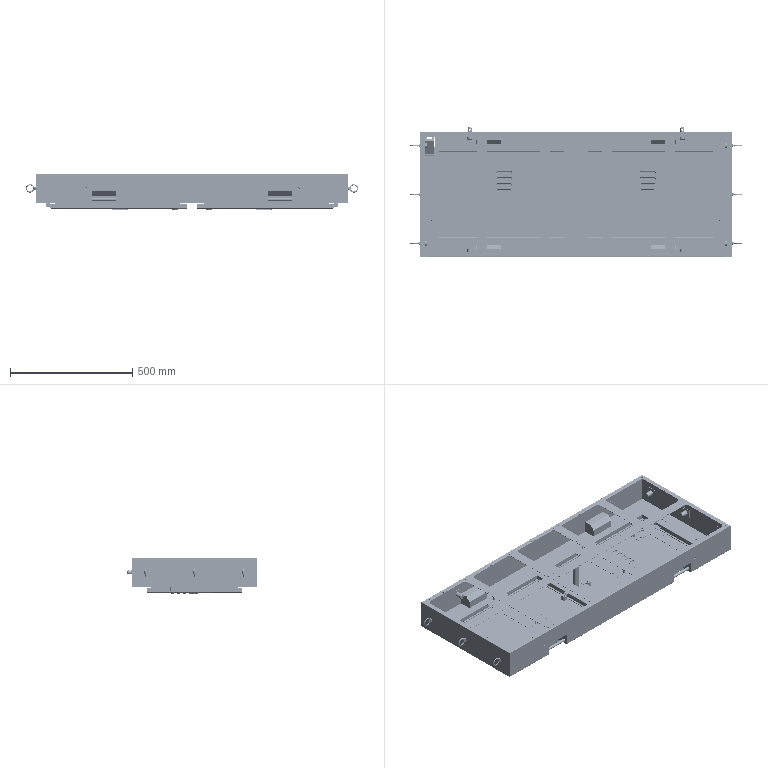Assembly | SolidWorks | mm | 99 component files | 197 solids | 6349 faces | box 1358.97 x 530.5 x 149.3 mm | volume 2529904 mm3 | plane 2960 | cylinder 2668 | spline 465 | cone 132 | torus 108 | sphere 16 | commonest cylinder face diameters 8 x438 9.619 x426 3 x332 5 x208 6 x184 9 x160 0.2 x132 4 x112
Bill of materials:
CL203-2-B | 4 |  | Rectangular block with rounded vertical edges and small edge rounds or chamfers, and two round holes in the top face, one near each end.
ControlCardMountingPlate | 1 |  | Thin flat rectangular plate with four short cylindrical bosses on one face and four smaller plain holes.
CL203-2-A | 4 |  | Rectangular block with rounded edges and a single cylindrical pin with a rounded tip sticking out of one face.
LeftDoorPanel | 1 |  | Shallow rectangular tray or pan with a thin base, a short upturned wall around the edge, a group of five parallel slots with rounded ends, one larger hole with flat sides, and small holes in one side wall.
LouverSupplement | 10 |  | Long, thin-walled, open half-shell or trough with rounded ends and a curved cross-section, like a capsule shape cut in half lengthwise.
Lock(MS407) | 2 |  | Short octagonal body sitting on a wider round flange with a conical underside. A small square boss with a center hole stands on the top face.
LockPlate | 2 |  | Flat strip with full-radius ends and a joggle (offset bend) partway along its length. A square through hole sits near one end.
WaterproofRubberStrip | 2 | BUTYL | Very thin, flat, rectangular frame (an outline shape with a large rectangular opening in the middle).
M10LiftingEye | 6 |  | Eye-type fitting: a round ring (torus) joined through a collar with a conical seat to a straight threaded shank.
M10LocatingPin | 2 |  | Turned part with a threaded shank, a short relief neck, and a larger cylindrical head with a chamfered end and a through hole running across it.
BoxSupport | 1 |  | Long, straight U-channel (C-shaped) profile with constant wall thickness and rounded inside and outside bends.
BSO-M3-10 | 2 |  | Cylindrical shank with a thin hexagonal flange or head at one end.
BSO-M3-20 | 12 |  | Plain cylindrical shank with a thin, wider hexagonal head at one end; the far end is flat.
CableTie | 19 |  | Constant-thickness strip bent into a hat (omega) profile: a raised flat crown, two sloped webs and two flat outer flanges, all with rounded bends.
Handle(Latest) | 4 |  | Sheet-metal bracket with a flat top panel and two folded-down end panels. The end panels have one chamfered corner. A solid cylindrical rod runs between the end panels below the top panel, and the bottom is open.
InletHole(New) | 1 |  | Sheet-metal piece bent into a triangular, tent-like prism with two flat outward flanges at the base. There is one round hole on the upper surface.
M10WaterproofStud | 10 |  | Solid stepped cylinder: a larger-diameter main body with a chamfered end edge and a shorter, smaller coaxial boss at the other end.
M10WaterproofStudWeldment | 10 |  | Flat square plate with a large central circular through-hole and four small circular through-holes near the corners.
M3RivetNut | 1 |  | Many very small, separate point-like bodies scattered in a regular grid-like pattern. There is no continuous solid shape.
P16Box | 1 |  | Large rectangular open frame or tray: perimeter walls surround a top grid of flat crossbars that form many rectangular openings. Small holes are spread along the bars, and there are round holes and rectangular notches in the walls.
Stiffener | 1 | AISI 1020 Steel, Cold Rolled | Grid of thin, slender bars: one long bar with four evenly spaced perpendicular bars crossing it.
PowerSupplyMountingPlate | 2 |  | Thin rectangular flat plate with four short cylindrical bosses near the corners, each with a centre hole, plus four small through-holes near the short edges.
RightDoorPanel | 1 |  | Shallow rectangular tray or cover: a flat panel with a low upturned flange around the edge. It has five parallel rounded-end slots, one rounded-square hole, and small holes in one flange.
Mates:
1. coincident | P16BoxWeldment-1/P16Box-1 face at (-69.394, 13.542, -50.6) dir (0, 0, -1) | CL203-2-B-1 face at (513.608, -116.478, -50.6) dir (0, 0, 1)
2. concentric | P16BoxWeldment-1/P16Box-1 edge at (520.108, -92.228, -50.6) dir (0, 0, -1) r 2.75 | CL203-2-B-1 edge at (520.108, -92.228, -50.6) dir (0, 0, 1) r 2.5
3. concentric | P16BoxWeldment-1/P16Box-1 edge at (520.108, -111.228, -49.4) dir (0, 0, -1) r 2.75 | CL203-2-B-1 edge at (520.108, -111.228, -50.6) dir (0, 0, 1) r 2.5
4. coincident | P16BoxWeldment-1/P16Box-1 face at (-69.394, 13.542, -50.6) dir (0, 0, -1) | CL203-2-B-2 face at (513.608, 81.062, -50.6) dir (0, 0, 1)
5. concentric | P16BoxWeldment-1/P16Box-1 edge at (520.108, 105.312, -50.6) dir (0, 0, -1) r 2.75 | CL203-2-B-2 edge at (520.108, 105.312, -50.6) dir (0, 0, 1) r 2.5
6. concentric | P16BoxWeldment-1/P16Box-1 edge at (520.108, 86.312, -49.4) dir (0, 0, -1) r 2.75 | CL203-2-B-2 edge at (520.108, 86.312, -50.6) dir (0, 0, 1) r 2.5
7. coincident | P16BoxWeldment-1/P16Box-1 face at (-69.394, 13.542, -50.6) dir (0, 0, -1) | CL203-2-B-3 face at (-665.396, 81.062, -50.6) dir (0, 0, 1)
8. concentric | P16BoxWeldment-1/P16Box-1 edge at (-658.896, 105.312, -50.6) dir (0, 0, -1) r 2.75 | CL203-2-B-3 edge at (-658.896, 105.312, -50.6) dir (0, 0, 1) r 2.5
9. concentric | P16BoxWeldment-1/P16Box-1 edge at (-658.896, 86.312, -49.4) dir (0, 0, -1) r 2.75 | CL203-2-B-3 edge at (-658.896, 86.312, -50.6) dir (0, 0, 1) r 2.5
10. coincident | P16BoxWeldment-1/P16Box-1 face at (-69.394, 13.542, -50.6) dir (0, 0, -1) | CL203-2-B-4 face at (-665.396, -116.478, -50.6) dir (0, 0, 1)
11. concentric | P16BoxWeldment-1/P16Box-1 edge at (-658.896, -92.228, -50.6) dir (0, 0, -1) r 2.75 | CL203-2-B-4 edge at (-658.896, -92.228, -50.6) dir (0, 0, 1) r 2.5
12. concentric | P16BoxWeldment-1/P16Box-1 edge at (-658.896, -111.228, -49.4) dir (0, 0, -1) r 2.75 | CL203-2-B-4 edge at (-658.896, -111.228, -50.6) dir (0, 0, 1) r 2.5
13. coincident | P16BoxWeldment-1/P16Box-1 face at (-69.394, 268.792, 68.2) dir (0, 1, 0) | M10LocatingPin-1 face at (370.106, 268.792, 9.4) dir (0, -1, 0)
14. concentric | P16BoxWeldment-1/M10WaterproofNutWeldment-2/M10WaterproofStud-1 edge at (365.606, 268.792, 9.4) dir (0, -1, 0) r 6.85 | M10LocatingPin-1 edge at (365.606, 285.292, 9.4) dir (0, -1, 0) r 8
15. coincident | P16BoxWeldment-1/P16Box-1 face at (-69.394, 268.792, 68.2) dir (0, 1, 0) | M10LocatingPin-3 face at (-499.894, 268.792, 9.4) dir (0, -1, 0)
16. concentric | P16BoxWeldment-1/M10WaterproofNutWeldment-1/M10WaterproofStud-1 edge at (-504.394, 268.792, 9.4) dir (0, -1, 0) r 5.3 | M10LocatingPin-3 edge at (-504.394, 285.292, 9.4) dir (0, -1, 0) r 8
17. concentric | CL203-2-B-1 edge at (520.108, -85.478, -60.6) dir (0, -1, 0) r 3.25 | LeftDoorPanelAssembly-1/CL203-2-A-1 edge at (520.108, -98.478, -60.6) dir (0, 1, 0) r 2.5
18. coincident | CL203-2-B-1 face at (527.608, -85.478, -50.6) dir (0, 1, 0) | LeftDoorPanelAssembly-1/CL203-2-A-1 face at (510.108, -85.478, -53.1) dir (0, -1, 0)
19. concentric | CL203-2-B-4 edge at (-658.896, -85.478, -60.6) dir (0, -1, 0) r 3.25 | RightDoorPanelAssembly-1/CL203-2-A-1 edge at (-658.896, -98.478, -60.6) dir (0, 1, 0) r 2.5
20. coincident | CL203-2-B-4 face at (-651.396, -85.478, -50.6) dir (0, 1, 0) | RightDoorPanelAssembly-1/CL203-2-A-1 face at (-648.896, -85.478, -68.1) dir (0, -1, 0)
21. coincident | P16BoxWeldment-1/BSO-M3-20-17 face at (46.106, 91.707, 49.4) dir (0, 0, -1) | PowerSupplyMountingPlate-3 face at (113.731, -28.293, 49.4) dir (0, 0, 1)
22. concentric | P16BoxWeldment-1/BSO-M3-20-17 edge at (46.106, 91.707, 49.4) dir (0, 0, -1) r 1.5 | PowerSupplyMountingPlate-3 edge at (46.106, 91.707, 48.2) dir (0, 0, 1) r 2
23. concentric | P16BoxWeldment-1/BSO-M3-20-18 edge at (71.106, 91.707, 49.4) dir (0, 0, -1) r 1.5 | PowerSupplyMountingPlate-3 edge at (71.106, 91.707, 48.2) dir (0, 0, 1) r 2
24. coincident | P16BoxWeldment-1/BSO-M3-20-17 face at (46.106, 91.707, 49.4) dir (0, 0, -1) | PowerSupplyMountingPlate-4 face at (-398.269, -28.293, 49.4) dir (0, 0, 1)
25. concentric | P16BoxWeldment-1/BSO-M3-20-13 edge at (-465.894, 91.707, 49.4) dir (0, 0, -1) r 1.5 | PowerSupplyMountingPlate-4 edge at (-465.894, 91.707, 48.2) dir (0, 0, 1) r 2
26. concentric | P16BoxWeldment-1/BSO-M3-20-14 edge at (-440.894, 91.707, 49.4) dir (0, 0, -1) r 1.5 | PowerSupplyMountingPlate-4 edge at (-440.894, 91.707, 48.2) dir (0, 0, 1) r 2
27. coincident | P16BoxWeldment-1/BSO-M3-20-23 face at (374.606, 26.042, 49.4) dir (0, 0, -1) | ControlCardMountingPlate-1 face at (314.606, 56.042, 49.4) dir (0, 0, 1)
28. concentric | P16BoxWeldment-1/BSO-M3-20-23 edge at (374.606, 26.042, 49.4) dir (0, 0, -1) r 2.7 | ControlCardMountingPlate-1 edge at (374.606, 26.042, 48.2) dir (0, 0, -1) r 2
29. concentric | P16BoxWeldment-1/BSO-M3-20-24 edge at (374.606, 1.042, 49.4) dir (0, 0, -1) r 2.7 | ControlCardMountingPlate-1 edge at (374.606, 1.042, 48.2) dir (0, 0, -1) r 2
30. coincident | P16BoxWeldment-1/P16Box-1 face at (-708.644, 13.542, 68.2) dir (-1, 0, 0) | M10LiftingEye-1 face at (-708.644, 213.542, 9.4) dir (1, 0, 0)
31. concentric | P16BoxWeldment-1/M10WaterproofNutWeldment-7/M10WaterproofStud-1 edge at (-708.544, 213.542, 9.4) dir (1, 0, 0) r 6.95 | M10LiftingEye-1 edge at (-708.644, 213.542, 9.4) dir (1, 0, 0) r 5.5
32. coincident | P16BoxWeldment-1/P16Box-1 face at (-708.644, 13.542, 68.2) dir (-1, 0, 0) | M10LiftingEye-2 face at (-708.644, 13.542, 9.4) dir (1, 0, 0)
33. concentric | P16BoxWeldment-1/M10WaterproofNutWeldment-8/M10WaterproofStud-1 edge at (-708.644, 13.542, 9.4) dir (1, 0, 0) r 5.3 | M10LiftingEye-2 edge at (-708.644, 13.542, 9.4) dir (1, 0, 0) r 5.5
34. coincident | P16BoxWeldment-1/P16Box-1 face at (-708.644, 13.542, 68.2) dir (-1, 0, 0) | M10LiftingEye-3 face at (-708.644, -186.458, 9.4) dir (1, 0, 0)
35. concentric | P16BoxWeldment-1/M10WaterproofNutWeldment-9/M10WaterproofStud-1 edge at (-708.644, -186.458, 9.4) dir (1, 0, 0) r 5.3 | M10LiftingEye-3 edge at (-708.644, -186.458, 9.4) dir (1, 0, 0) r 5.5
36. coincident | P16BoxWeldment-1/P16Box-1 face at (569.856, 13.542, 68.2) dir (1, 0, 0) | M10LiftingEye-4 face at (569.856, 213.542, 9.4) dir (-1, 0, 0)
37. concentric | P16BoxWeldment-1/M10WaterproofNutWeldment-12/M10WaterproofStud-1 edge at (569.756, 213.542, 9.4) dir (-1, 0, 0) r 6.95 | M10LiftingEye-4 edge at (569.856, 213.542, 9.4) dir (-1, 0, 0) r 5.5
38. coincident | P16BoxWeldment-1/P16Box-1 face at (569.856, 13.542, 68.2) dir (1, 0, 0) | M10LiftingEye-5 face at (569.856, 13.542, 9.4) dir (-1, 0, 0)
39. concentric | P16BoxWeldment-1/M10WaterproofNutWeldment-11/M10WaterproofStud-1 edge at (569.756, 13.542, 9.4) dir (-1, 0, 0) r 6.95 | M10LiftingEye-5 edge at (569.856, 13.542, 9.4) dir (-1, 0, 0) r 5.5
40. coincident | P16BoxWeldment-1/P16Box-1 face at (569.856, 13.542, 68.2) dir (1, 0, 0) | M10LiftingEye-6 face at (569.856, -186.458, 9.4) dir (-1, 0, 0)
41. concentric | P16BoxWeldment-1/M10WaterproofNutWeldment-10/M10WaterproofStud-1 edge at (569.756, -186.458, 9.4) dir (-1, 0, 0) r 6.95 | M10LiftingEye-6 edge at (569.856, -186.458, 9.4) dir (-1, 0, 0) r 5.5
42. coincident | LeftDoorPanelAssembly-1/LeftDoorPanelWeldment-1/LeftDoorPanel-1 face at (230.358, 13.542, -73.1) dir (0, 0, -1) | RightDoorPanelAssembly-1/RightDoorPanelWeldment-1/RightDoorPanel-1 face at (-369.146, 227.042, -73.1) dir (0, 0, -1)
43. coincident | LeftDoorPanelWeldment-1/LeftDoorPanel-1 face at (-299.618, -4.448, 10) dir (-1, 0, 0) | CL203-2-A-1 face at (-299.618, -72.468, 4) dir (1, 0, 0)
44. concentric | LeftDoorPanelWeldment-1/LeftDoorPanel-1 edge at (-298.418, -77.718, -2.5) dir (-1, 0, 0) r 2.75 | CL203-2-A-1 edge at (-299.618, -77.718, -2.5) dir (1, 0, 0) r 2.5
45. concentric | LeftDoorPanelWeldment-1/LeftDoorPanel-1 edge at (-298.418, -96.718, -2.5) dir (-1, 0, 0) r 2.75 | CL203-2-A-1 edge at (-299.618, -96.718, -2.5) dir (1, 0, 0) r 2.5
46. coincident | LeftDoorPanelWeldment-1/LeftDoorPanel-1 face at (-299.618, -4.448, 10) dir (-1, 0, 0) | CL203-2-A-2 face at (-299.618, 125.072, 4) dir (1, 0, 0)
47. concentric | LeftDoorPanelWeldment-1/LeftDoorPanel-1 edge at (-299.618, 119.822, -2.5) dir (-1, 0, 0) r 2.75 | CL203-2-A-2 edge at (-299.618, 119.822, -2.5) dir (1, 0, 0) r 2.5
48. concentric | LeftDoorPanelWeldment-1/LeftDoorPanel-1 edge at (-298.418, 100.822, -2.5) dir (-1, 0, 0) r 2.75 | CL203-2-A-2 edge at (-299.618, 100.822, -2.5) dir (1, 0, 0) r 2.5
49. coincident | LeftDoorPanelWeldment-1/LeftDoorPanel-1 face at (-19.868, -4.448, 10) dir (0, 0, 1) | Lock(MS407)-1 face at (209.879, -4.448, 10) dir (0, 0, -1)
50. concentric | LeftDoorPanelWeldment-1/LeftDoorPanel-1 edge at (209.879, -4.448, 8.8) dir (0, 0, 1) r 11.35 | Lock(MS407)-1 edge at (209.879, -4.448, -9) dir (0, 0, -1) r 11.25
51. parallel | LeftDoorPanelWeldment-1/LeftDoorPanel-1 edge at (214.608, 5.87, 8.8) dir (-1, 0, 0) | Lock(MS407)-1 face at (204.823, 5.602, -9) dir (0, 1, 0)
52. coincident | Lock(MS407)-1 face at (209.879, -4.448, -9) dir (0, 0, -1) | LockPlate-1 face at (199.879, -12.448, -9) dir (0, 0, 1)
53. coincident | Lock(MS407)-1 face at (205.879, -8.448, -12) dir (-1, 0, 0) | LockPlate-1 face at (205.879, -0.4485, -19) dir (1, 0, 0)
54. coincident | Lock(MS407)-1 face at (205.879, -0.4485, -12) dir (0, 1, 0) | LockPlate-1 face at (205.879, -0.4485, -19) dir (0, -1, 0)
55. coincident | LeftDoorPanelWeldment-1/LeftDoorPanel-1 face at (-19.868, -4.448, 8.8) dir (0, 0, -1) | WaterproofRubberStrip-1 face at (-24.868, -4.448, 8.8) dir (0, 0, 1)
56. coincident | LeftDoorPanelWeldment-1/LeftDoorPanel-1 face at (-19.868, 189.852, 10) dir (0, -1, 0) | WaterproofRubberStrip-1 face at (248.682, 189.852, 8.8) dir (0, 1, 0)
57. coincident | LeftDoorPanelWeldment-1/LeftDoorPanel-1 face at (-298.418, -4.448, 10) dir (1, 0, 0) | WaterproofRubberStrip-1 face at (-298.418, -198.748, 8.8) dir (-1, 0, 0)
58. parallel | LeftDoorPanel-1 face at (-49.524, 215.963, 10) dir (0, 1, 0) | LouverSupplement-5 face at (-78.502, 5.963, 16.8) dir (0, -1, 0)
59. concentric | LeftDoorPanel-1 edge at (-68.502, 7.963, 10) dir (0, 0, 1) r 10 | LouverSupplement-5 edge at (-68.502, 7.963, 10) dir (0, 0, -1) r 10
60. coincident | LeftDoorPanel-1 face at (-49.524, 20.463, 8.8) dir (0, 0, -1) | LouverSupplement-5 face at (-68.502, 7.963, 8.8) dir (0, 0, -1)
61. parallel | LeftDoorPanel-1 face at (-49.524, 215.963, 10) dir (0, 1, 0) | LouverSupplement-12 face at (-78.502, 30.963, 16.8) dir (0, -1, 0)
62. coincident | LeftDoorPanel-1 face at (-49.524, 20.463, 8.8) dir (0, 0, -1) | LouverSupplement-12 face at (-68.502, 32.963, 8.8) dir (0, 0, -1)
63. concentric | LeftDoorPanel-1 edge at (-68.502, 32.963, 10) dir (0, 0, 1) r 10 | LouverSupplement-12 edge at (-68.502, 32.963, 10) dir (0, 0, -1) r 10
64. parallel | LeftDoorPanel-1 face at (-49.524, 215.963, 10) dir (0, 1, 0) | LouverSupplement-13 face at (-78.502, 55.963, 16.8) dir (0, -1, 0)
65. concentric | LeftDoorPanel-1 edge at (-68.502, 57.963, 10) dir (0, 0, 1) r 10 | LouverSupplement-13 edge at (-68.502, 57.963, 10) dir (0, 0, -1) r 10
66. coincident | LeftDoorPanel-1 face at (-49.524, 20.463, 8.8) dir (0, 0, -1) | LouverSupplement-13 face at (-68.502, 57.963, 8.8) dir (0, 0, -1)
67. parallel | LeftDoorPanel-1 face at (-49.524, 215.963, 10) dir (0, 1, 0) | LouverSupplement-14 face at (-78.502, 80.963, 16.8) dir (0, -1, 0)
68. concentric | LeftDoorPanel-1 edge at (-68.502, 82.963, 10) dir (0, 0, 1) r 10 | LouverSupplement-14 edge at (-68.502, 82.963, 10) dir (0, 0, -1) r 10
69. coincident | LeftDoorPanel-1 face at (-49.524, 20.463, 8.8) dir (0, 0, -1) | LouverSupplement-14 face at (-68.502, 82.963, 8.8) dir (0, 0, -1)
70. parallel | LeftDoorPanel-1 face at (-49.524, 215.963, 10) dir (0, 1, 0) | LouverSupplement-15 face at (-78.502, 105.963, 16.8) dir (0, -1, 0)
71. concentric | LeftDoorPanel-1 edge at (-68.502, 107.963, 10) dir (0, 0, 1) r 10 | LouverSupplement-15 edge at (-68.502, 107.963, 10) dir (0, 0, -1) r 10
72. coincident | LeftDoorPanel-1 face at (-49.524, 20.463, 8.8) dir (0, 0, -1) | LouverSupplement-15 face at (-68.502, 107.963, 8.8) dir (0, 0, -1)
73. coincident | P16Box-1 face at (-68.504, 34.698, 68.2) dir (0, 0, -1) | Stiffener-1 face at (-68.504, 28.198, 68.2) dir (0, 0, 1)
74. distance | P16Box-1 face at (-68.504, -220.552, 68.2) dir (0, -1, 0) | Stiffener-1 face at (52.996, -218.052, 68.2) dir (0, -1, 0)
75. distance | P16Box-1 face at (-707.754, 34.698, 68.2) dir (-1, 0, 0) | Stiffener-1 face at (-705.254, 28.198, 68.2) dir (-1, 0, 0)
76. coincident | P16Box-1 face at (-68.504, 288.748, 68.2) dir (0, -1, 0) | M10WaterproofNutWeldment-1/M10WaterproofStudWeldment-1 face at (-503.504, 288.748, 9.4) dir (0, 1, 0)
77. concentric | P16Box-1 edge at (-503.504, 289.948, 9.4) dir (0, 1, 0) r 7 | M10WaterproofNutWeldment-1/M10WaterproofStud-1 edge at (-503.504, 289.848, 9.4) dir (0, -1, 0) r 6.95
78. coincident | P16Box-1 face at (-68.504, 288.748, 68.2) dir (0, -1, 0) | M10WaterproofNutWeldment-2/M10WaterproofStudWeldment-1 face at (366.496, 288.748, 9.4) dir (0, 1, 0)
79. concentric | P16Box-1 edge at (366.496, 288.748, 9.4) dir (0, 1, 0) r 7 | M10WaterproofNutWeldment-2/M10WaterproofStud-1 edge at (366.496, 289.848, 9.4) dir (0, -1, 0) r 6.95
80. parallel | P16Box-1 face at (-68.504, 34.698, 69.4) dir (0, 0, 1) | M10WaterproofNutWeldment-2/M10WaterproofStudWeldment-1 face at (346.996, 286.748, 28.9) dir (0, 0, 1)
81. parallel | P16Box-1 face at (-68.504, 34.698, 69.4) dir (0, 0, 1) | M10WaterproofNutWeldment-1/M10WaterproofStudWeldment-1 face at (-523.004, 286.748, 28.9) dir (0, 0, 1)
82. coincident | P16Box-1 face at (-68.504, -220.552, 68.2) dir (0, -1, 0) | BSO-M3-10-1 face at (286.496, -220.552, 9.4) dir (0, -1, 0)
83. coincident | P16Box-1 face at (-68.504, -220.552, 68.2) dir (0, -1, 0) | BSO-M3-10-2 face at (-423.504, -220.552, 9.4) dir (0, -1, 0)
84. coincident | P16Box-1 face at (-68.504, -219.352, 68.2) dir (0, 1, 0) | CableTie-1 face at (-439.754, -219.352, 13.4) dir (0, -1, 0)
85. distance | CableTie-1 face at (-443.046, -219.352, 9.4) dir (0, 0, -1) | P16Box-1 face at (-68.504, 34.698, -50.6) dir (0, 0, -1)
86. distance | CableTie-1 face at (-457.754, -219.352, 13.4) dir (-1, 0, 0) | P16Box-1 face at (-707.754, 34.698, 68.2) dir (-1, 0, 0)
87. coincident | Stiffener-1 face at (-68.504, 28.198, 61.2) dir (0, 0, -1) | CableTie-3 face at (-574.004, 36.698, 61.2) dir (0, 0, 1)
88. distance | CableTie-3 face at (-588.712, 32.698, 60.1) dir (0, -1, 0) | Stiffener-1 face at (-705.254, 28.198, 68.2) dir (0, -1, 0)
89. distance | CableTie-3 face at (-574.004, 36.698, 60.2) dir (1, 0, 0) | Stiffener-1 face at (-459.004, 41.198, 68.2) dir (-1, 0, 0)
90. coincident | Stiffener-1 face at (-68.504, 28.198, 61.2) dir (0, 0, -1) | CableTie-4 face at (-318.004, 36.698, 61.2) dir (0, 0, 1)
91. distance | CableTie-4 face at (-332.712, 32.698, 60.1) dir (0, -1, 0) | Stiffener-1 face at (-705.254, 28.198, 68.2) dir (0, -1, 0)
92. distance | CableTie-4 face at (-318.004, 36.698, 60.2) dir (1, 0, 0) | Stiffener-1 face at (-203.004, 41.198, 68.2) dir (-1, 0, 0)
93. coincident | Stiffener-1 face at (-68.504, 28.198, 61.2) dir (0, 0, -1) | CableTie-6 face at (193.996, 36.698, 61.2) dir (0, 0, 1)
94. distance | CableTie-6 face at (179.288, 32.698, 60.1) dir (0, -1, 0) | Stiffener-1 face at (-705.254, 28.198, 68.2) dir (0, -1, 0)
95. distance | CableTie-6 face at (193.996, 36.698, 60.2) dir (1, 0, 0) | Stiffener-1 face at (308.996, 41.198, 68.2) dir (-1, 0, 0)
96. coincident | Stiffener-1 face at (-68.504, 28.198, 61.2) dir (0, 0, -1) | CableTie-7 face at (454.546, 36.698, 61.2) dir (0, 0, 1)
97. distance | CableTie-7 face at (439.838, 32.698, 60.1) dir (0, -1, 0) | Stiffener-1 face at (-705.254, 28.198, 68.2) dir (0, -1, 0)
98. distance | CableTie-7 face at (454.546, 36.698, 60.2) dir (1, 0, 0) | P16Box-1 face at (569.546, 34.698, 68.2) dir (-1, 0, 0)
99. coincident | CableTie-4 face at (-331.004, 36.698, 55.7) dir (0, 0, -1) | CableTie-8 face at (-95.004, 36.698, 55.7) dir (0, 0, -1)
100. coincident | CableTie-4 face at (-332.712, 36.698, 60.1) dir (0, 1, 0) | CableTie-8 face at (-86.33, 36.698, 60.476) dir (0, 1, 0)
101. distance | CableTie-8 face at (-100.004, 36.698, 61.2) dir (-1, 0, 0) | Stiffener-1 face at (-190.004, 41.198, 68.2) dir (1, 0, 0)
102. coincident | CableTie-3 face at (-587.004, 36.698, 55.7) dir (0, 0, -1) | CableTie-9 face at (-454.504, -169.802, 55.7) dir (0, 0, -1)
103. distance | Stiffener-1 face at (-459.004, -218.052, 68.2) dir (-1, 0, 0) | CableTie-9 face at (-454.504, -171.51, 61.2) dir (-1, 0, 0)
104. distance | CableTie-9 face at (-454.504, -156.802, 60.2) dir (0, 1, 0) | Stiffener-1 face at (-446.004, 28.198, 68.2) dir (0, -1, 0)
105. coincident | P16Box-1 face at (-68.504, 34.698, -49.4) dir (0, 0, 1) | BoxSupport-1 face at (-77.004, 29.798, -49.4) dir (0, 0, -1)
106. distance | BoxSupport-1 face at (-58.504, 41.198, 61.2) dir (1, 0, 0) | P16Box-1 face at (-18.504, 34.698, 68.2) dir (1, 0, 0)
107. coincident | Stiffener-1 face at (-190.004, 28.198, 68.2) dir (0, -1, 0) | BoxSupport-1 face at (-78.504, 28.198, 61.2) dir (0, -1, 0)
108. coincident | P16Box-1 face at (-706.554, 34.698, 68.2) dir (1, 0, 0) | M10WaterproofNutWeldment-7/M10WaterproofStudWeldment-1 face at (-706.554, 234.698, 9.4) dir (-1, 0, 0)
109. concentric | P16Box-1 edge at (-706.554, 234.698, 9.4) dir (-1, 0, 0) r 7 | M10WaterproofNutWeldment-7/M10WaterproofStud-1 edge at (-677.554, 234.698, 9.4) dir (1, 0, 0) r 10
110. parallel | P16Box-1 face at (-68.504, 34.698, -50.6) dir (0, 0, -1) | M10WaterproofNutWeldment-7/M10WaterproofStudWeldment-1 face at (-704.554, 254.198, -10.1) dir (0, 0, -1)
111. coincident | P16Box-1 face at (-706.554, 34.698, 68.2) dir (1, 0, 0) | M10WaterproofNutWeldment-8/M10WaterproofStudWeldment-1 face at (-706.554, 34.698, 9.4) dir (-1, 0, 0)
112. parallel | P16Box-1 face at (-68.504, 34.698, -50.6) dir (0, 0, -1) | M10WaterproofNutWeldment-8/M10WaterproofStudWeldment-1 face at (-704.554, 54.198, -10.1) dir (0, 0, -1)
113. concentric | P16Box-1 edge at (-706.554, 34.698, 9.4) dir (-1, 0, 0) r 7 | M10WaterproofNutWeldment-8/M10WaterproofStud-1 edge at (-677.554, 34.698, 9.4) dir (1, 0, 0) r 10
114. coincident | P16Box-1 face at (-706.554, 34.698, 68.2) dir (1, 0, 0) | M10WaterproofNutWeldment-9/M10WaterproofStudWeldment-1 face at (-706.554, -165.302, 9.4) dir (-1, 0, 0)
115. concentric | P16Box-1 edge at (-706.554, -165.302, 9.4) dir (-1, 0, 0) r 7 | M10WaterproofNutWeldment-9/M10WaterproofStud-1 edge at (-677.554, -165.302, 9.4) dir (1, 0, 0) r 10
116. parallel | P16Box-1 face at (-68.504, 34.698, -50.6) dir (0, 0, -1) | M10WaterproofNutWeldment-9/M10WaterproofStudWeldment-1 face at (-704.554, -145.802, -10.1) dir (0, 0, -1)
117. coincident | P16Box-1 face at (569.546, 34.698, 68.2) dir (-1, 0, 0) | M10WaterproofNutWeldment-10/M10WaterproofStudWeldment-1 face at (569.546, -165.302, 9.4) dir (1, 0, 0)
118. concentric | P16Box-1 edge at (569.546, -165.302, 9.4) dir (1, 0, 0) r 7 | M10WaterproofNutWeldment-10/M10WaterproofStud-1 edge at (540.546, -165.302, 9.4) dir (-1, 0, 0) r 10
119. parallel | P16Box-1 face at (-68.504, 34.698, 69.4) dir (0, 0, 1) | M10WaterproofNutWeldment-10/M10WaterproofStudWeldment-1 face at (567.546, -145.802, 28.9) dir (0, 0, 1)
120. coincident | P16Box-1 face at (569.546, 34.698, 68.2) dir (-1, 0, 0) | M10WaterproofNutWeldment-11/M10WaterproofStudWeldment-1 face at (569.546, 34.698, 9.4) dir (1, 0, 0)
121. parallel | P16Box-1 face at (-68.504, 34.698, 69.4) dir (0, 0, 1) | M10WaterproofNutWeldment-11/M10WaterproofStudWeldment-1 face at (567.546, 54.198, 28.9) dir (0, 0, 1)
122. concentric | P16Box-1 edge at (569.546, 34.698, 9.4) dir (1, 0, 0) r 7 | M10WaterproofNutWeldment-11/M10WaterproofStud-1 edge at (540.546, 34.698, 9.4) dir (-1, 0, 0) r 10
123. coincident | P16Box-1 face at (569.546, 34.698, 68.2) dir (-1, 0, 0) | M10WaterproofNutWeldment-12/M10WaterproofStudWeldment-1 face at (569.546, 234.698, 9.4) dir (1, 0, 0)
124. concentric | P16Box-1 edge at (569.546, 234.698, 9.4) dir (1, 0, 0) r 7 | M10WaterproofNutWeldment-12/M10WaterproofStud-1 edge at (540.546, 234.698, 9.4) dir (-1, 0, 0) r 10
125. parallel | P16Box-1 face at (-68.504, 34.698, 69.4) dir (0, 0, 1) | M10WaterproofNutWeldment-12/M10WaterproofStudWeldment-1 face at (567.546, 254.198, 28.9) dir (0, 0, 1)
126. coincident | P16Box-1 face at (-68.504, -219.352, 68.2) dir (0, 1, 0) | M10WaterproofNutWeldment-13/M10WaterproofStudWeldment-1 face at (366.496, -219.352, 9.4) dir (0, -1, 0)
127. concentric | P16Box-1 edge at (366.496, -219.352, 9.4) dir (0, -1, 0) r 7 | M10WaterproofNutWeldment-13/M10WaterproofStud-1 edge at (366.496, -190.352, 9.4) dir (0, 1, 0) r 10
128. parallel | P16Box-1 face at (-68.504, 34.698, 68.2) dir (0, 0, -1) | M10WaterproofNutWeldment-13/M10WaterproofStudWeldment-1 face at (385.996, -217.352, 28.9) dir (0, 0, 1)
129. coincident | P16Box-1 face at (-68.504, -219.352, 68.2) dir (0, 1, 0) | M10WaterproofNutWeldment-14/M10WaterproofStudWeldment-1 face at (-503.504, -219.352, 9.4) dir (0, -1, 0)
130. parallel | P16Box-1 face at (-68.504, 34.698, 68.2) dir (0, 0, -1) | M10WaterproofNutWeldment-14/M10WaterproofStudWeldment-1 face at (-484.004, -217.352, 28.9) dir (0, 0, 1)
131. concentric | P16Box-1 edge at (-503.504, -219.352, 9.4) dir (0, -1, 0) r 7 | M10WaterproofNutWeldment-14/M10WaterproofStud-1 edge at (-503.504, -190.352, 9.4) dir (0, 1, 0) r 10
132. coincident | P16Box-1 face at (-68.504, 34.698, 69.4) dir (0, 0, 1) | BSO-M3-20-13 face at (-465.004, 112.864, 69.4) dir (0, 0, 1)
133. coincident | P16Box-1 face at (-68.504, 34.698, 69.4) dir (0, 0, 1) | BSO-M3-20-14 face at (-440.004, 112.864, 69.4) dir (0, 0, 1)
134. coincident | P16Box-1 face at (-68.504, 34.698, 69.4) dir (0, 0, 1) | BSO-M3-20-15 face at (-465.004, -127.136, 69.4) dir (0, 0, 1)
135. coincident | P16Box-1 face at (-68.504, 34.698, 69.4) dir (0, 0, 1) | BSO-M3-20-16 face at (-440.004, -127.136, 69.4) dir (0, 0, 1)
136. coincident | P16Box-1 face at (-68.504, 34.698, 69.4) dir (0, 0, 1) | BSO-M3-20-17 face at (46.996, 112.864, 69.4) dir (0, 0, 1)
137. coincident | P16Box-1 face at (-68.504, 34.698, 69.4) dir (0, 0, 1) | BSO-M3-20-18 face at (71.996, 112.864, 69.4) dir (0, 0, 1)
138. coincident | P16Box-1 face at (-68.504, 34.698, 69.4) dir (0, 0, 1) | BSO-M3-20-19 face at (46.996, -127.136, 69.4) dir (0, 0, 1)
139. coincident | P16Box-1 face at (-68.504, 34.698, 69.4) dir (0, 0, 1) | BSO-M3-20-20 face at (71.996, -127.136, 69.4) dir (0, 0, 1)
140. coincident | P16Box-1 face at (-68.504, 34.698, 69.4) dir (0, 0, 1) | BSO-M3-20-21 face at (255.496, 47.198, 69.4) dir (0, 0, 1)
141. coincident | P16Box-1 face at (-68.504, 34.698, 69.4) dir (0, 0, 1) | BSO-M3-20-22 face at (255.496, 22.198, 69.4) dir (0, 0, 1)
142. coincident | P16Box-1 face at (-68.504, 34.698, 69.4) dir (0, 0, 1) | BSO-M3-20-23 face at (375.496, 47.198, 69.4) dir (0, 0, 1)
143. coincident | P16Box-1 face at (-68.504, 34.698, 69.4) dir (0, 0, 1) | BSO-M3-20-24 face at (375.496, 22.198, 69.4) dir (0, 0, 1)
144. coincident | P16Box-1 face at (-68.504, 34.698, 68.2) dir (0, 0, -1) | M3RivetNut-1 face at (-692.504, 276.698, 68.2) dir (0, 0, 1)
145. concentric | P16Box-1 edge at (-692.504, 276.698, 69.4) dir (0, 0, 1) r 2.5 | M3RivetNut-1 edge at (-692.504, 276.698, 68.2) dir (0, 0, 1) r 1.5
146. concentric | P16Box-1 edge at (-596.504, 276.698, 69.4) dir (0, 0, 1) r 2.5 | M3RivetNut-1 edge at (-596.504, 276.698, 68.2) dir (0, 0, 1) r 3
147. coincident | P16Box-1 face at (-68.504, -219.352, 68.2) dir (0, 1, 0) | Handle(Latest)-2 face at (239.242, -219.352, -47.4) dir (0, -1, 0)
148. coincident | P16Box-1 face at (-68.504, 34.698, -2.4) dir (0, 0, -1) | Handle(Latest)-2 face at (342.246, -220.852, -2.4) dir (0, 0, -1)
149. coincident | P16Box-1 face at (240.746, -268.752, -2.4) dir (1, 0, 0) | Handle(Latest)-2 face at (240.746, -217.852, -47.9) dir (1, 0, 0)
150. coincident | P16Box-1 face at (-68.504, 34.698, -2.4) dir (0, 0, -1) | Handle(Latest)-4 face at (-376.254, -220.852, -2.4) dir (0, 0, -1)
151. coincident | P16Box-1 face at (-377.754, -172.352, -2.4) dir (0, -1, 0) | Handle(Latest)-4 face at (-376.254, -172.352, -19.285) dir (0, -1, 0)
152. coincident | P16Box-1 face at (-477.754, -268.752, -2.4) dir (1, 0, 0) | Handle(Latest)-4 face at (-477.754, -217.852, -47.9) dir (1, 0, 0)
153. coincident | P16Box-1 face at (240.746, 241.748, -2.4) dir (0, 1, 0) | Handle(Latest)-5 face at (239.246, 241.748, -19.285) dir (0, 1, 0)
154. coincident | P16Box-1 face at (-68.504, 34.698, -2.4) dir (0, 0, -1) | Handle(Latest)-5 face at (239.246, 290.248, -2.4) dir (0, 0, -1)
155. coincident | P16Box-1 face at (240.746, 338.148, -2.4) dir (1, 0, 0) | Handle(Latest)-5 face at (240.746, 287.248, -47.9) dir (1, 0, 0)
156. coincident | P16Box-1 face at (240.746, 241.748, -2.4) dir (0, 1, 0) | Handle(Latest)-6 face at (-479.254, 241.748, -19.285) dir (0, 1, 0)
157. coincident | P16Box-1 face at (-68.504, 34.698, -2.4) dir (0, 0, -1) | Handle(Latest)-6 face at (-479.254, 290.248, -2.4) dir (0, 0, -1)
158. coincident | P16Box-1 face at (-477.754, 338.148, -2.4) dir (1, 0, 0) | Handle(Latest)-6 face at (-477.754, 287.248, -47.9) dir (1, 0, 0)
159. coincident | P16Box-1 face at (-68.504, 34.698, -50.6) dir (0, 0, -1) | InletHole(New)-1 face at (-687.754, 276.848, -50.6) dir (0, 0, -1)
160. distance | InletHole(New)-1 face at (-687.754, 255.709, -15.442) dir (-1, 0, 0) | P16Box-1 face at (-687.904, 194.048, -49.4) dir (1, 0, 0)
161. distance | InletHole(New)-1 face at (-687.754, 283.848, -50.6) dir (0, 1, 0) | P16Box-1 face at (-687.904, 283.948, -49.4) dir (0, -1, 0)
162. concentric | P16Box-1 edge at (286.496, -219.352, 9.4) dir (0, -1, 0) r 2.7 | BSO-M3-10-1 edge at (286.496, -209.552, 9.4) dir (0, 1, 0) r 2.7
163. concentric | P16Box-1 edge at (-423.504, -219.352, 9.4) dir (0, -1, 0) r 2.7 | BSO-M3-10-2 edge at (-423.504, -209.552, 9.4) dir (0, 1, 0) r 2.7
164. concentric | P16Box-1 edge at (-465.004, 112.864, 68.2) dir (0, 0, 1) r 2.7 | BSO-M3-20-13 edge at (-465.004, 112.864, 49.4) dir (0, 0, -1) r 2.7
165. concentric | P16Box-1 edge at (-440.004, 112.864, 68.2) dir (0, 0, 1) r 2.7 | BSO-M3-20-14 edge at (-440.004, 112.864, 49.4) dir (0, 0, -1) r 2.7
166. concentric | P16Box-1 edge at (-465.004, -127.136, 68.2) dir (0, 0, 1) r 2.7 | BSO-M3-20-15 edge at (-465.004, -127.136, 49.4) dir (0, 0, -1) r 2.7
167. concentric | P16Box-1 edge at (-440.004, -127.136, 68.2) dir (0, 0, 1) r 2.7 | BSO-M3-20-16 edge at (-440.004, -127.136, 49.4) dir (0, 0, -1) r 2.7
168. concentric | P16Box-1 edge at (46.996, 112.864, 68.2) dir (0, 0, 1) r 2.7 | BSO-M3-20-17 edge at (46.996, 112.864, 49.4) dir (0, 0, -1) r 2.7
169. concentric | P16Box-1 edge at (71.996, 112.864, 68.2) dir (0, 0, 1) r 2.7 | BSO-M3-20-18 edge at (71.996, 112.864, 49.4) dir (0, 0, -1) r 2.7
170. concentric | P16Box-1 edge at (46.996, -127.136, 68.2) dir (0, 0, 1) r 2.7 | BSO-M3-20-19 edge at (46.996, -127.136, 49.4) dir (0, 0, -1) r 2.7
171. concentric | P16Box-1 edge at (71.996, -127.136, 68.2) dir (0, 0, 1) r 2.7 | BSO-M3-20-20 edge at (71.996, -127.136, 49.4) dir (0, 0, -1) r 2.7
172. concentric | P16Box-1 edge at (255.496, 47.198, 68.2) dir (0, 0, 1) r 2.7 | BSO-M3-20-21 edge at (255.496, 47.198, 49.4) dir (0, 0, -1) r 2.7
173. concentric | P16Box-1 edge at (255.496, 22.198, 68.2) dir (0, 0, 1) r 2.7 | BSO-M3-20-22 edge at (255.496, 22.198, 49.4) dir (0, 0, -1) r 2.7
174. concentric | P16Box-1 edge at (375.496, 47.198, 68.2) dir (0, 0, 1) r 2.7 | BSO-M3-20-23 edge at (375.496, 47.198, 49.4) dir (0, 0, -1) r 2.7
175. concentric | P16Box-1 edge at (375.496, 22.198, 68.2) dir (0, 0, 1) r 2.7 | BSO-M3-20-24 edge at (375.496, 22.198, 49.4) dir (0, 0, -1) r 2.7
176. coincident | M10WaterproofStudWeldment-1 face at (-61.09, 14.235, -1) dir (0, 0, -1) | M10WaterproofStud-1 face at (-60.35, 24.208, -1) dir (0, 0, 1)
177. concentric | M10WaterproofStudWeldment-1 edge at (-61.09, 14.235, 1) dir (0, 0, 1) r 7 | M10WaterproofStud-1 edge at (-61.09, 14.235, -1) dir (0, 0, -1) r 10
178. coincident | RightDoorPanelWeldment-1/RightDoorPanel-1 face at (-312.963, 215.279, -287.748) dir (-1, 0, 0) | CL203-2-A-1 face at (-312.963, -66.241, 9.002) dir (1, 0, 0)
179. concentric | RightDoorPanelWeldment-1/RightDoorPanel-1 edge at (-311.763, -90.491, 2.502) dir (1, 0, 0) r 2.75 | CL203-2-A-1 edge at (-312.963, -90.491, 2.502) dir (1, 0, 0) r 2.5
180. concentric | RightDoorPanelWeldment-1/RightDoorPanel-1 edge at (-311.763, -71.491, 2.502) dir (1, 0, 0) r 2.75 | CL203-2-A-1 edge at (-312.963, -71.491, 2.502) dir (1, 0, 0) r 2.5
181. coincident | RightDoorPanelWeldment-1/RightDoorPanel-1 face at (-312.963, 215.279, -287.748) dir (-1, 0, 0) | CL203-2-A-2 face at (-312.963, 131.299, 9.002) dir (1, 0, 0)
182. concentric | RightDoorPanelWeldment-1/RightDoorPanel-1 edge at (-311.763, 107.049, 2.502) dir (1, 0, 0) r 2.75 | CL203-2-A-2 edge at (-312.963, 107.049, 2.502) dir (1, 0, 0) r 2.5
183. concentric | RightDoorPanelWeldment-1/RightDoorPanel-1 edge at (-311.763, 126.049, 2.502) dir (1, 0, 0) r 2.75 | CL203-2-A-2 edge at (-312.963, 126.049, 2.502) dir (1, 0, 0) r 2.5
184. concentric | RightDoorPanelWeldment-1/RightDoorPanel-1 edge at (196.534, 1.779, -9.998) dir (0, 0, 1) r 11.25 | Lock(MS407)-1 edge at (196.534, 1.779, 9.002) dir (0, 0, 1) r 11.25
185. coincident | RightDoorPanelWeldment-1/RightDoorPanel-1 face at (-33.213, 215.279, -9.998) dir (0, 0, -1) | Lock(MS407)-1 face at (196.534, 1.779, -9.998) dir (0, 0, 1)
186. parallel | RightDoorPanelWeldment-1/RightDoorPanel-1 face at (246.537, 215.279, -287.748) dir (1, 0, 0) | Lock(MS407)-1 face at (206.584, -3.276, 9.002) dir (1, 0, 0)
187. coincident | Lock(MS407)-1 face at (196.534, 1.779, 9.002) dir (0, 0, 1) | LockPlate-1 face at (186.534, 9.779, 9.002) dir (0, 0, -1)
188. coincident | Lock(MS407)-1 face at (192.534, -2.221, 12.002) dir (-1, 0, 0) | LockPlate-1 face at (192.534, -2.221, 19.002) dir (1, 0, 0)
189. coincident | Lock(MS407)-1 face at (200.534, 5.779, 12.002) dir (0, 1, 0) | LockPlate-1 face at (192.534, 5.779, 19.002) dir (0, -1, 0)
190. coincident | RightDoorPanelWeldment-1/RightDoorPanel-1 face at (-33.213, 215.279, -8.798) dir (0, 0, 1) | WaterproofRubberStrip-1 face at (-38.213, 1.779, -8.798) dir (0, 0, -1)
191. coincident | RightDoorPanelWeldment-1/RightDoorPanel-1 face at (-33.213, 196.079, 10.002) dir (0, -1, 0) | WaterproofRubberStrip-1 face at (235.337, 196.079, -6.298) dir (0, 1, 0)
192. coincident | RightDoorPanelWeldment-1/RightDoorPanel-1 face at (-311.763, 215.279, -287.748) dir (1, 0, 0) | WaterproofRubberStrip-1 face at (-311.763, -192.521, -6.298) dir (-1, 0, 0)
193. coincident | RightDoorPanel-1 face at (-46.262, 217.652, -8.798) dir (0, 0, 1) | LouverSupplement-1 face at (-15.24, 91.652, -8.798) dir (0, 0, 1)
194. parallel | RightDoorPanel-1 face at (-46.262, 199.652, 10.002) dir (0, 1, 0) | LouverSupplement-1 face at (-5.24, 89.652, -16.798) dir (0, -1, 0)
195. concentric | RightDoorPanel-1 edge at (-15.24, 91.652, -9.998) dir (0, 0, 1) r 10 | LouverSupplement-1 edge at (-15.24, 91.652, -9.998) dir (0, 0, 1) r 10
196. coincident | RightDoorPanel-1 face at (-46.262, 217.652, -8.798) dir (0, 0, 1) | LouverSupplement-2 face at (-15.24, 66.652, -8.798) dir (0, 0, 1)
197. parallel | RightDoorPanel-1 face at (-46.262, 199.652, 10.002) dir (0, 1, 0) | LouverSupplement-2 face at (-5.24, 64.652, -16.798) dir (0, -1, 0)
198. concentric | RightDoorPanel-1 edge at (-15.24, 66.652, -9.998) dir (0, 0, 1) r 10 | LouverSupplement-2 edge at (-15.24, 66.652, -9.998) dir (0, 0, 1) r 10
199. coincident | RightDoorPanel-1 face at (-46.262, 217.652, -8.798) dir (0, 0, 1) | LouverSupplement-3 face at (-15.24, 41.652, -8.798) dir (0, 0, 1)
200. parallel | RightDoorPanel-1 face at (-46.262, 199.652, 10.002) dir (0, 1, 0) | LouverSupplement-3 face at (-5.24, 39.652, -16.798) dir (0, -1, 0)
201. concentric | RightDoorPanel-1 edge at (-15.24, 41.652, -9.998) dir (0, 0, 1) r 10 | LouverSupplement-3 edge at (-15.24, 41.652, -9.998) dir (0, 0, 1) r 10
202. coincident | RightDoorPanel-1 face at (-46.262, 217.652, -8.798) dir (0, 0, 1) | LouverSupplement-4 face at (-15.24, 16.652, -8.798) dir (0, 0, 1)
203. parallel | RightDoorPanel-1 face at (-46.262, 199.652, 10.002) dir (0, 1, 0) | LouverSupplement-4 face at (-5.24, 14.652, -16.798) dir (0, -1, 0)
204. concentric | RightDoorPanel-1 edge at (-15.24, 16.652, -9.998) dir (0, 0, 1) r 10 | LouverSupplement-4 edge at (-15.24, 16.652, -9.998) dir (0, 0, 1) r 10
205. coincident | RightDoorPanel-1 face at (-46.262, 217.652, -8.798) dir (0, 0, 1) | LouverSupplement-5 face at (-15.24, -8.348, -8.798) dir (0, 0, 1)
206. parallel | RightDoorPanel-1 face at (-46.262, 199.652, 10.002) dir (0, 1, 0) | LouverSupplement-5 face at (-5.24, -10.348, -16.798) dir (0, -1, 0)
207. concentric | RightDoorPanel-1 edge at (-15.24, -8.348, -9.998) dir (0, 0, 1) r 10 | LouverSupplement-5 edge at (-15.24, -8.348, -9.998) dir (0, 0, 1) r 10